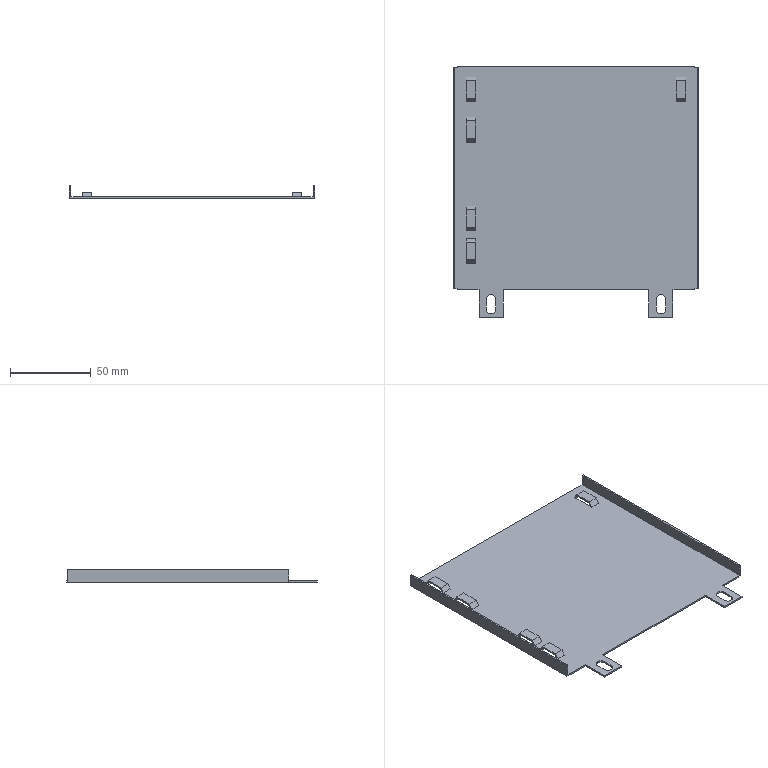Component | NX | BOTTOM_PANEL | 1 solid | 84 faces | volume 23364 mm3 | plane 80 | cylinder 4 | commonest cylinder face diameters 6 x4